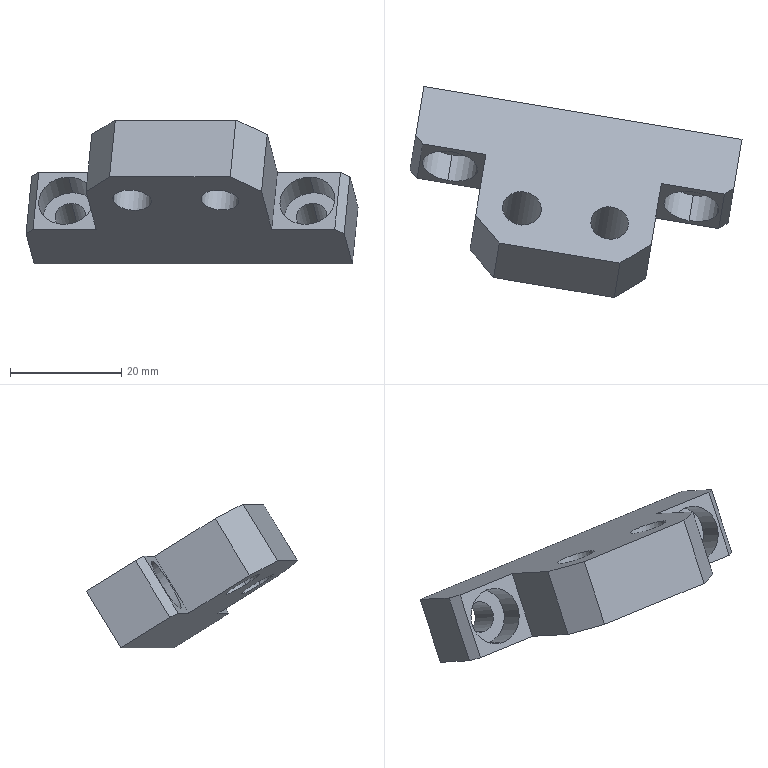Component | SolidWorks | 14AC-24-1-014-1 | 1 solid | 28 faces | box 59.71 x 37.99 x 25.9 mm | volume 12878 mm3 | plane 16 | cylinder 12 | commonest cylinder face diameters 10 x4 5.5 x4 6.8 x2 7 x2
build123d program:
from build123d import *

# Parameters (mm, degrees)
BOSS_EXTRUDE1_DEPTH                             = 12
M8X1_0_TAPPED_HOLE1_D                           = 7
CHAMFER1_SIZE                                   = 5
M5_HEX_SOCKET_HEAD_CAP_SCREW_CBORE1_D           = 5.5
M5_HEX_SOCKET_HEAD_CAP_SCREW_CBORE1_CBORE_D     = 10
M5_HEX_SOCKET_HEAD_CAP_SCREW_CBORE1_CBORE_DEPTH = 5.4
CHAMFER2_SIZE                                   = 1.5
M8_TAPPED_HOLE1_D                               = 6.8
M8_TAPPED_HOLE1_DEPTH                           = 19.75
M8_TAPPED_HOLE1_TIP                             = 2.043


with BuildPart() as part:
    # Sketch1 → Boss-Extrude1 (new body)
    with BuildSketch(Plane.XY):
        Polygon((-16, 0), (-16, 18), (16, 18), (16, 0), (29, 0), (29, -12), (-29, -12), (-29, 0), align=None)
    extrude(amount=BOSS_EXTRUDE1_DEPTH)

    # M8x1.0 Tapped Hole1 (through all)
    with Locations(Plane(origin=(-8, 10, 12), x_dir=(1, 0, 0), z_dir=(0, 0, 1))):
        with Locations((0, 0)):
            Hole(M8X1_0_TAPPED_HOLE1_D / 2)

    # Chamfer1
    chamfer1_edges = [part.edges().sort_by_distance(p)[0] for p in [
        (-16, 18, 6),
        (16, 18, 6),
    ]]
    chamfer(chamfer1_edges, length=CHAMFER1_SIZE)

    # M5 Hex Socket Head Cap Screw CBORE1 (through all)
    with Locations(Plane(origin=(-22, 0, 6), x_dir=(0, 0, 1), z_dir=(0, 1, 0))):
        with Locations((0, 0), (0, 44)):
            CounterBoreHole(M5_HEX_SOCKET_HEAD_CAP_SCREW_CBORE1_D / 2, M5_HEX_SOCKET_HEAD_CAP_SCREW_CBORE1_CBORE_D / 2, M5_HEX_SOCKET_HEAD_CAP_SCREW_CBORE1_CBORE_DEPTH)

    # Chamfer2
    chamfer2_edges = [part.edges().sort_by_distance(p)[0] for p in [
        (29, 0, 6),
        (-29, 0, 6),
    ]]
    chamfer(chamfer2_edges, length=CHAMFER2_SIZE)

    # M8 Tapped Hole1
    with Locations(Plane(origin=(8, 10, 12), x_dir=(1, 0, 0), z_dir=(0, 0, 1))):
        with Locations((0, 0)):
            Hole(M8_TAPPED_HOLE1_D / 2, depth=M8_TAPPED_HOLE1_DEPTH)
            with Locations((0, 0, -(M8_TAPPED_HOLE1_DEPTH + M8_TAPPED_HOLE1_TIP / 2))):  # 118° drill point
                Cone(0, M8_TAPPED_HOLE1_D / 2, M8_TAPPED_HOLE1_TIP, mode=Mode.SUBTRACT)


solid = part.part

# Placed as in the assembly
solid = solid.moved(Location((416.585, -110.808, -130.095), (148.871, -4.92, 8.082)))
STEP:
#1=COLOUR_RGB('',0.7922,0.8196,0.9333);
#2=FILL_AREA_STYLE_COLOUR('',#1);
#3=FILL_AREA_STYLE('',(#2));
#4=SURFACE_STYLE_FILL_AREA(#3);
#5=SURFACE_SIDE_STYLE('',(#4));
#6=SURFACE_STYLE_USAGE(.BOTH.,#5);
#7=PRESENTATION_STYLE_ASSIGNMENT((#6));
#8=CARTESIAN_POINT('',(16.524,-4.723,-4.916));
#9=VERTEX_POINT('',#8);
#10=CARTESIAN_POINT('',(16.789,-4.767,-4.916));
#11=VERTEX_POINT('',#10);
#12=CARTESIAN_POINT('',(16.657,-4.745,-4.916));
#13=DIRECTION('',(-0.08576,-0.5151,-0.8529));
#14=DIRECTION('',(0.9864,-0.1642,0.));
#15=AXIS2_PLACEMENT_3D('',#12,#13,#14);
#16=CIRCLE('',#15,0.1339);
#17=EDGE_CURVE('',#9,#11,#16,.T.);
#18=ORIENTED_EDGE('',*,*,#17,.F.);
#19=CARTESIAN_POINT('',(16.484,-4.967,-5.319));
#20=VERTEX_POINT('',#19);
#21=CARTESIAN_POINT('',(16.484,-4.967,-5.319));
#22=DIRECTION('',(-0.08576,-0.5151,-0.8529));
#23=VECTOR('',#22,39.37);
#24=LINE('',#21,#23);
#25=EDGE_CURVE('',#9,#20,#24,.T.);
#26=ORIENTED_EDGE('',*,*,#25,.T.);
#27=CARTESIAN_POINT('',(16.748,-5.011,-5.319));
#28=VERTEX_POINT('',#27);
#29=CARTESIAN_POINT('',(16.616,-4.989,-5.319));
#30=DIRECTION('',(-0.08576,-0.5151,-0.8529));
#31=DIRECTION('',(0.9864,-0.1642,0.));
#32=AXIS2_PLACEMENT_3D('',#29,#30,#31);
#33=CIRCLE('',#32,0.1339);
#34=EDGE_CURVE('',#20,#28,#33,.T.);
#35=ORIENTED_EDGE('',*,*,#34,.T.);
#36=CARTESIAN_POINT('',(16.748,-5.011,-5.319));
#37=DIRECTION('',(-0.08576,-0.5151,-0.8529));
#38=VECTOR('',#37,39.37);
#39=LINE('',#36,#38);
#40=EDGE_CURVE('',#11,#28,#39,.T.);
#41=ORIENTED_EDGE('',*,*,#40,.F.);
#42=EDGE_LOOP('',(#18,#26,#35,#41));
#43=FACE_OUTER_BOUND('',#42,.T.);
#44=CARTESIAN_POINT('',(16.616,-4.989,-5.319));
#45=DIRECTION('',(-0.08576,-0.5151,-0.8529));
#46=DIRECTION('',(0.9864,-0.1642,0.));
#47=AXIS2_PLACEMENT_3D('',#44,#45,#46);
#48=CYLINDRICAL_SURFACE('',#47,0.1339);
#49=ADVANCED_FACE('',(#43),#48,.F.);
#50=CARTESIAN_POINT('',(15.573,-4.062,-5.266));
#51=VERTEX_POINT('',#50);
#52=CARTESIAN_POINT('',(15.539,-4.264,-5.602));
#53=VERTEX_POINT('',#52);
#54=CARTESIAN_POINT('',(15.556,-4.163,-5.434));
#55=DIRECTION('',(-0.1401,-0.8413,0.5222));
#56=DIRECTION('',(-0.08576,-0.5151,-0.8529));
#57=AXIS2_PLACEMENT_3D('',#54,#55,#56);
#58=CIRCLE('',#57,0.1969);
#59=EDGE_CURVE('',#51,#53,#58,.T.);
#60=ORIENTED_EDGE('',*,*,#59,.F.);
#61=CARTESIAN_POINT('',(15.543,-4.241,-5.155));
#62=VERTEX_POINT('',#61);
#63=CARTESIAN_POINT('',(15.543,-4.241,-5.155));
#64=DIRECTION('',(-0.1401,-0.8413,0.5222));
#65=VECTOR('',#64,39.37);
#66=LINE('',#63,#65);
#67=EDGE_CURVE('',#51,#62,#66,.T.);
#68=ORIENTED_EDGE('',*,*,#67,.T.);
#69=CARTESIAN_POINT('',(15.509,-4.443,-5.491));
#70=VERTEX_POINT('',#69);
#71=CARTESIAN_POINT('',(15.526,-4.342,-5.323));
#72=DIRECTION('',(-0.1401,-0.8413,0.5222));
#73=DIRECTION('',(-0.08576,-0.5151,-0.8529));
#74=AXIS2_PLACEMENT_3D('',#71,#72,#73);
#75=CIRCLE('',#74,0.1969);
#76=EDGE_CURVE('',#62,#70,#75,.T.);
#77=ORIENTED_EDGE('',*,*,#76,.T.);
#78=CARTESIAN_POINT('',(15.509,-4.443,-5.491));
#79=DIRECTION('',(-0.1401,-0.8413,0.5222));
#80=VECTOR('',#79,39.37);
#81=LINE('',#78,#80);
#82=EDGE_CURVE('',#53,#70,#81,.T.);
#83=ORIENTED_EDGE('',*,*,#82,.F.);
#84=EDGE_LOOP('',(#60,#68,#77,#83));
#85=FACE_OUTER_BOUND('',#84,.T.);
#86=CARTESIAN_POINT('',(15.526,-4.342,-5.323));
#87=DIRECTION('',(-0.1401,-0.8413,0.5222));
#88=DIRECTION('',(-0.08576,-0.5151,-0.8529));
#89=AXIS2_PLACEMENT_3D('',#86,#87,#88);
#90=CYLINDRICAL_SURFACE('',#89,0.1969);
#91=ADVANCED_FACE('',(#85),#90,.F.);
#92=CARTESIAN_POINT('',(15.602,-3.889,-5.478));
#93=VERTEX_POINT('',#92);
#94=CARTESIAN_POINT('',(15.583,-4.,-5.662));
#95=VERTEX_POINT('',#94);
#96=CARTESIAN_POINT('',(15.593,-3.944,-5.57));
#97=DIRECTION('',(-0.1401,-0.8413,0.5222));
#98=DIRECTION('',(-0.08576,-0.5151,-0.8529));
#99=AXIS2_PLACEMENT_3D('',#96,#97,#98);
#100=CIRCLE('',#99,0.1083);
#101=EDGE_CURVE('',#93,#95,#100,.T.);
#102=ORIENTED_EDGE('',*,*,#101,.F.);
#103=CARTESIAN_POINT('',(15.565,-4.107,-5.342));
#104=VERTEX_POINT('',#103);
#105=CARTESIAN_POINT('',(15.536,-4.286,-5.231));
#106=DIRECTION('',(-0.1401,-0.8413,0.5222));
#107=VECTOR('',#106,39.37);
#108=LINE('',#105,#107);
#109=EDGE_CURVE('',#93,#104,#108,.T.);
#110=ORIENTED_EDGE('',*,*,#109,.T.);
#111=CARTESIAN_POINT('',(15.547,-4.219,-5.527));
#112=VERTEX_POINT('',#111);
#113=CARTESIAN_POINT('',(15.556,-4.163,-5.434));
#114=DIRECTION('',(-0.1401,-0.8413,0.5222));
#115=DIRECTION('',(-0.08576,-0.5151,-0.8529));
#116=AXIS2_PLACEMENT_3D('',#113,#114,#115);
#117=CIRCLE('',#116,0.1083);
#118=EDGE_CURVE('',#104,#112,#117,.T.);
#119=ORIENTED_EDGE('',*,*,#118,.T.);
#120=CARTESIAN_POINT('',(15.517,-4.398,-5.416));
#121=DIRECTION('',(-0.1401,-0.8413,0.5222));
#122=VECTOR('',#121,39.37);
#123=LINE('',#120,#122);
#124=EDGE_CURVE('',#95,#112,#123,.T.);
#125=ORIENTED_EDGE('',*,*,#124,.F.);
#126=EDGE_LOOP('',(#102,#110,#119,#125));
#127=FACE_OUTER_BOUND('',#126,.T.);
#128=CARTESIAN_POINT('',(15.526,-4.342,-5.323));
#129=DIRECTION('',(-0.1401,-0.8413,0.5222));
#130=DIRECTION('',(-0.08576,-0.5151,-0.8529));
#131=AXIS2_PLACEMENT_3D('',#128,#129,#130);
#132=CYLINDRICAL_SURFACE('',#131,0.1083);
#133=ADVANCED_FACE('',(#127),#132,.F.);
#134=CARTESIAN_POINT('',(17.282,-4.346,-5.266));
#135=VERTEX_POINT('',#134);
#136=CARTESIAN_POINT('',(17.248,-4.549,-5.602));
#137=VERTEX_POINT('',#136);
#138=CARTESIAN_POINT('',(17.265,-4.448,-5.434));
#139=DIRECTION('',(-0.1401,-0.8413,0.5222));
#140=DIRECTION('',(-0.08576,-0.5151,-0.8529));
#141=AXIS2_PLACEMENT_3D('',#138,#139,#140);
#142=CIRCLE('',#141,0.1969);
#143=EDGE_CURVE('',#135,#137,#142,.T.);
#144=ORIENTED_EDGE('',*,*,#143,.F.);
#145=CARTESIAN_POINT('',(17.252,-4.525,-5.155));
#146=VERTEX_POINT('',#145);
#147=CARTESIAN_POINT('',(17.252,-4.525,-5.155));
#148=DIRECTION('',(-0.1401,-0.8413,0.5222));
#149=VECTOR('',#148,39.37);
#150=LINE('',#147,#149);
#151=EDGE_CURVE('',#135,#146,#150,.T.);
#152=ORIENTED_EDGE('',*,*,#151,.T.);
#153=CARTESIAN_POINT('',(17.218,-4.728,-5.491));
#154=VERTEX_POINT('',#153);
#155=CARTESIAN_POINT('',(17.235,-4.626,-5.323));
#156=DIRECTION('',(-0.1401,-0.8413,0.5222));
#157=DIRECTION('',(-0.08576,-0.5151,-0.8529));
#158=AXIS2_PLACEMENT_3D('',#155,#156,#157);
#159=CIRCLE('',#158,0.1969);
#160=EDGE_CURVE('',#146,#154,#159,.T.);
#161=ORIENTED_EDGE('',*,*,#160,.T.);
#162=CARTESIAN_POINT('',(17.218,-4.728,-5.491));
#163=DIRECTION('',(-0.1401,-0.8413,0.5222));
#164=VECTOR('',#163,39.37);
#165=LINE('',#162,#164);
#166=EDGE_CURVE('',#137,#154,#165,.T.);
#167=ORIENTED_EDGE('',*,*,#166,.F.);
#168=EDGE_LOOP('',(#144,#152,#161,#167));
#169=FACE_OUTER_BOUND('',#168,.T.);
#170=CARTESIAN_POINT('',(17.235,-4.626,-5.323));
#171=DIRECTION('',(-0.1401,-0.8413,0.5222));
#172=DIRECTION('',(-0.08576,-0.5151,-0.8529));
#173=AXIS2_PLACEMENT_3D('',#170,#171,#172);
#174=CYLINDRICAL_SURFACE('',#173,0.1969);
#175=ADVANCED_FACE('',(#169),#174,.F.);
#176=CARTESIAN_POINT('',(17.311,-4.173,-5.478));
#177=VERTEX_POINT('',#176);
#178=CARTESIAN_POINT('',(17.292,-4.285,-5.662));
#179=VERTEX_POINT('',#178);
#180=CARTESIAN_POINT('',(17.301,-4.229,-5.57));
#181=DIRECTION('',(-0.1401,-0.8413,0.5222));
#182=DIRECTION('',(-0.08576,-0.5151,-0.8529));
#183=AXIS2_PLACEMENT_3D('',#180,#181,#182);
#184=CIRCLE('',#183,0.1083);
#185=EDGE_CURVE('',#177,#179,#184,.T.);
#186=ORIENTED_EDGE('',*,*,#185,.F.);
#187=CARTESIAN_POINT('',(17.274,-4.392,-5.342));
#188=VERTEX_POINT('',#187);
#189=CARTESIAN_POINT('',(17.244,-4.571,-5.231));
#190=DIRECTION('',(-0.1401,-0.8413,0.5222));
#191=VECTOR('',#190,39.37);
#192=LINE('',#189,#191);
#193=EDGE_CURVE('',#177,#188,#192,.T.);
#194=ORIENTED_EDGE('',*,*,#193,.T.);
#195=CARTESIAN_POINT('',(17.256,-4.503,-5.527));
#196=VERTEX_POINT('',#195);
#197=CARTESIAN_POINT('',(17.265,-4.448,-5.434));
#198=DIRECTION('',(-0.1401,-0.8413,0.5222));
#199=DIRECTION('',(-0.08576,-0.5151,-0.8529));
#200=AXIS2_PLACEMENT_3D('',#197,#198,#199);
#201=CIRCLE('',#200,0.1083);
#202=EDGE_CURVE('',#188,#196,#201,.T.);
#203=ORIENTED_EDGE('',*,*,#202,.T.);
#204=CARTESIAN_POINT('',(17.226,-4.682,-5.416));
#205=DIRECTION('',(-0.1401,-0.8413,0.5222));
#206=VECTOR('',#205,39.37);
#207=LINE('',#204,#206);
#208=EDGE_CURVE('',#179,#196,#207,.T.);
#209=ORIENTED_EDGE('',*,*,#208,.F.);
#210=EDGE_LOOP('',(#186,#194,#203,#209));
#211=FACE_OUTER_BOUND('',#210,.T.);
#212=CARTESIAN_POINT('',(17.235,-4.626,-5.323));
#213=DIRECTION('',(-0.1401,-0.8413,0.5222));
#214=DIRECTION('',(-0.08576,-0.5151,-0.8529));
#215=AXIS2_PLACEMENT_3D('',#212,#213,#214);
#216=CYLINDRICAL_SURFACE('',#215,0.1083);
#217=ADVANCED_FACE('',(#211),#216,.F.);
#218=CARTESIAN_POINT('',(15.899,-4.619,-4.916));
#219=VERTEX_POINT('',#218);
#220=CARTESIAN_POINT('',(16.171,-4.665,-4.916));
#221=VERTEX_POINT('',#220);
#222=CARTESIAN_POINT('',(16.035,-4.642,-4.916));
#223=DIRECTION('',(-0.08576,-0.5151,-0.8529));
#224=DIRECTION('',(0.9864,-0.1642,0.));
#225=AXIS2_PLACEMENT_3D('',#222,#223,#224);
#226=CIRCLE('',#225,0.1378);
#227=EDGE_CURVE('',#219,#221,#226,.T.);
#228=ORIENTED_EDGE('',*,*,#227,.F.);
#229=CARTESIAN_POINT('',(15.859,-4.863,-5.319));
#230=VERTEX_POINT('',#229);
#231=CARTESIAN_POINT('',(15.859,-4.863,-5.319));
#232=DIRECTION('',(-0.08576,-0.5151,-0.8529));
#233=VECTOR('',#232,39.37);
#234=LINE('',#231,#233);
#235=EDGE_CURVE('',#219,#230,#234,.T.);
#236=ORIENTED_EDGE('',*,*,#235,.T.);
#237=CARTESIAN_POINT('',(16.131,-4.908,-5.319));
#238=VERTEX_POINT('',#237);
#239=CARTESIAN_POINT('',(15.995,-4.885,-5.319));
#240=DIRECTION('',(-0.08576,-0.5151,-0.8529));
#241=DIRECTION('',(0.9864,-0.1642,0.));
#242=AXIS2_PLACEMENT_3D('',#239,#240,#241);
#243=CIRCLE('',#242,0.1378);
#244=EDGE_CURVE('',#230,#238,#243,.T.);
#245=ORIENTED_EDGE('',*,*,#244,.T.);
#246=CARTESIAN_POINT('',(16.131,-4.908,-5.319));
#247=DIRECTION('',(-0.08576,-0.5151,-0.8529));
#248=VECTOR('',#247,39.37);
#249=LINE('',#246,#248);
#250=EDGE_CURVE('',#221,#238,#249,.T.);
#251=ORIENTED_EDGE('',*,*,#250,.F.);
#252=EDGE_LOOP('',(#228,#236,#245,#251));
#253=FACE_OUTER_BOUND('',#252,.T.);
#254=CARTESIAN_POINT('',(15.995,-4.885,-5.319));
#255=DIRECTION('',(-0.08576,-0.5151,-0.8529));
#256=DIRECTION('',(0.9864,-0.1642,0.));
#257=AXIS2_PLACEMENT_3D('',#254,#255,#256);
#258=CYLINDRICAL_SURFACE('',#257,0.1378);
#259=ADVANCED_FACE('',(#253),#258,.F.);
#260=CARTESIAN_POINT('',(15.526,-4.342,-5.323));
#261=DIRECTION('',(-0.1401,-0.8413,0.5222));
#262=DIRECTION('',(-0.08576,-0.5151,-0.8529));
#263=AXIS2_PLACEMENT_3D('',#260,#261,#262);
#264=CIRCLE('',#263,0.1969);
#265=EDGE_CURVE('',#70,#62,#264,.T.);
#266=ORIENTED_EDGE('',*,*,#265,.F.);
#267=ORIENTED_EDGE('',*,*,#76,.F.);
#268=EDGE_LOOP('',(#266,#267));
#269=FACE_BOUND('',#268,.T.);
#270=CARTESIAN_POINT('',(15.78,-4.259,-5.122));
#271=VERTEX_POINT('',#270);
#272=CARTESIAN_POINT('',(15.333,-4.185,-5.122));
#273=VERTEX_POINT('',#272);
#274=CARTESIAN_POINT('',(15.275,-4.175,-5.122));
#275=DIRECTION('',(-0.9864,0.1642,0.));
#276=VECTOR('',#275,39.37);
#277=LINE('',#274,#276);
#278=EDGE_CURVE('',#271,#273,#277,.T.);
#279=ORIENTED_EDGE('',*,*,#278,.T.);
#280=CARTESIAN_POINT('',(15.292,-4.428,-5.525));
#281=VERTEX_POINT('',#280);
#282=CARTESIAN_POINT('',(15.292,-4.428,-5.525));
#283=DIRECTION('',(-0.08576,-0.5151,-0.8529));
#284=VECTOR('',#283,39.37);
#285=LINE('',#282,#284);
#286=EDGE_CURVE('',#273,#281,#285,.T.);
#287=ORIENTED_EDGE('',*,*,#286,.T.);
#288=CARTESIAN_POINT('',(15.739,-4.502,-5.525));
#289=VERTEX_POINT('',#288);
#290=CARTESIAN_POINT('',(15.234,-4.418,-5.525));
#291=DIRECTION('',(-0.9864,0.1642,0.));
#292=VECTOR('',#291,39.37);
#293=LINE('',#290,#292);
#294=EDGE_CURVE('',#289,#281,#293,.T.);
#295=ORIENTED_EDGE('',*,*,#294,.F.);
#296=CARTESIAN_POINT('',(15.739,-4.502,-5.525));
#297=DIRECTION('',(0.08576,0.5151,0.8529));
#298=VECTOR('',#297,39.37);
#299=LINE('',#296,#298);
#300=EDGE_CURVE('',#289,#271,#299,.T.);
#301=ORIENTED_EDGE('',*,*,#300,.T.);
#302=EDGE_LOOP('',(#279,#287,#295,#301));
#303=FACE_OUTER_BOUND('',#302,.T.);
#304=CARTESIAN_POINT('',(15.234,-4.418,-5.525));
#305=DIRECTION('',(0.1401,0.8413,-0.5222));
#306=DIRECTION('',(0.08576,0.5151,0.8529));
#307=AXIS2_PLACEMENT_3D('',#304,#305,#306);
#308=PLANE('',#307);
#309=ADVANCED_FACE('',(#269,#303),#308,.F.);
#310=CARTESIAN_POINT('',(15.243,-4.369,-5.556));
#311=VERTEX_POINT('',#310);
#312=CARTESIAN_POINT('',(15.3,-4.021,-5.771));
#313=VERTEX_POINT('',#312);
#314=CARTESIAN_POINT('',(15.3,-4.021,-5.771));
#315=DIRECTION('',(0.1401,0.8413,-0.5222));
#316=VECTOR('',#315,39.37);
#317=LINE('',#314,#316);
#318=EDGE_CURVE('',#311,#313,#317,.T.);
#319=ORIENTED_EDGE('',*,*,#318,.F.);
#320=CARTESIAN_POINT('',(15.283,-4.125,-5.153));
#321=VERTEX_POINT('',#320);
#322=CARTESIAN_POINT('',(15.243,-4.369,-5.556));
#323=DIRECTION('',(0.08576,0.5151,0.8529));
#324=VECTOR('',#323,39.37);
#325=LINE('',#322,#324);
#326=EDGE_CURVE('',#311,#321,#325,.T.);
#327=ORIENTED_EDGE('',*,*,#326,.T.);
#328=CARTESIAN_POINT('',(15.341,-3.778,-5.369));
#329=VERTEX_POINT('',#328);
#330=CARTESIAN_POINT('',(15.341,-3.778,-5.369));
#331=DIRECTION('',(0.1401,0.8413,-0.5222));
#332=VECTOR('',#331,39.37);
#333=LINE('',#330,#332);
#334=EDGE_CURVE('',#321,#329,#333,.T.);
#335=ORIENTED_EDGE('',*,*,#334,.T.);
#336=CARTESIAN_POINT('',(15.3,-4.021,-5.771));
#337=DIRECTION('',(0.08576,0.5151,0.8529));
#338=VECTOR('',#337,39.37);
#339=LINE('',#336,#338);
#340=EDGE_CURVE('',#313,#329,#339,.T.);
#341=ORIENTED_EDGE('',*,*,#340,.F.);
#342=EDGE_LOOP('',(#319,#327,#335,#341));
#343=FACE_OUTER_BOUND('',#342,.T.);
#344=CARTESIAN_POINT('',(15.3,-4.021,-5.771));
#345=DIRECTION('',(0.9864,-0.1642,-0.));
#346=DIRECTION('',(0.08576,0.5151,0.8529));
#347=AXIS2_PLACEMENT_3D('',#344,#345,#346);
#348=PLANE('',#347);
#349=ADVANCED_FACE('',(#343),#348,.F.);
#350=CARTESIAN_POINT('',(15.593,-3.944,-5.57));
#351=DIRECTION('',(-0.1401,-0.8413,0.5222));
#352=DIRECTION('',(-0.08576,-0.5151,-0.8529));
#353=AXIS2_PLACEMENT_3D('',#350,#351,#352);
#354=CIRCLE('',#353,0.1083);
#355=EDGE_CURVE('',#95,#93,#354,.T.);
#356=ORIENTED_EDGE('',*,*,#355,.T.);
#357=ORIENTED_EDGE('',*,*,#101,.T.);
#358=EDGE_LOOP('',(#356,#357));
#359=FACE_BOUND('',#358,.T.);
#360=CARTESIAN_POINT('',(17.301,-4.229,-5.57));
#361=DIRECTION('',(-0.1401,-0.8413,0.5222));
#362=DIRECTION('',(-0.08576,-0.5151,-0.8529));
#363=AXIS2_PLACEMENT_3D('',#360,#361,#362);
#364=CIRCLE('',#363,0.1083);
#365=EDGE_CURVE('',#179,#177,#364,.T.);
#366=ORIENTED_EDGE('',*,*,#365,.T.);
#367=ORIENTED_EDGE('',*,*,#185,.T.);
#368=EDGE_LOOP('',(#366,#367));
#369=FACE_BOUND('',#368,.T.);
#370=CARTESIAN_POINT('',(17.593,-4.153,-5.369));
#371=VERTEX_POINT('',#370);
#372=CARTESIAN_POINT('',(17.593,-4.153,-5.369));
#373=DIRECTION('',(0.9864,-0.1642,-0.));
#374=VECTOR('',#373,39.37);
#375=LINE('',#372,#374);
#376=EDGE_CURVE('',#329,#371,#375,.T.);
#377=ORIENTED_EDGE('',*,*,#376,.T.);
#378=CARTESIAN_POINT('',(17.553,-4.396,-5.771));
#379=VERTEX_POINT('',#378);
#380=CARTESIAN_POINT('',(17.553,-4.396,-5.771));
#381=DIRECTION('',(0.08576,0.5151,0.8529));
#382=VECTOR('',#381,39.37);
#383=LINE('',#380,#382);
#384=EDGE_CURVE('',#379,#371,#383,.T.);
#385=ORIENTED_EDGE('',*,*,#384,.F.);
#386=CARTESIAN_POINT('',(17.553,-4.396,-5.771));
#387=DIRECTION('',(0.9864,-0.1642,-0.));
#388=VECTOR('',#387,39.37);
#389=LINE('',#386,#388);
#390=EDGE_CURVE('',#313,#379,#389,.T.);
#391=ORIENTED_EDGE('',*,*,#390,.F.);
#392=ORIENTED_EDGE('',*,*,#340,.T.);
#393=EDGE_LOOP('',(#377,#385,#391,#392));
#394=FACE_OUTER_BOUND('',#393,.T.);
#395=CARTESIAN_POINT('',(17.553,-4.396,-5.771));
#396=DIRECTION('',(-0.1401,-0.8413,0.5222));
#397=DIRECTION('',(-0.9864,0.1642,0.));
#398=AXIS2_PLACEMENT_3D('',#395,#396,#397);
#399=PLANE('',#398);
#400=ADVANCED_FACE('',(#359,#369,#394),#399,.F.);
#401=CARTESIAN_POINT('',(17.535,-4.5,-5.153));
#402=VERTEX_POINT('',#401);
#403=CARTESIAN_POINT('',(17.527,-4.55,-5.122));
#404=DIRECTION('',(-0.1401,-0.8413,0.5222));
#405=VECTOR('',#404,39.37);
#406=LINE('',#403,#405);
#407=EDGE_CURVE('',#371,#402,#406,.T.);
#408=ORIENTED_EDGE('',*,*,#407,.T.);
#409=CARTESIAN_POINT('',(17.495,-4.744,-5.556));
#410=VERTEX_POINT('',#409);
#411=CARTESIAN_POINT('',(17.495,-4.744,-5.556));
#412=DIRECTION('',(-0.08576,-0.5151,-0.8529));
#413=VECTOR('',#412,39.37);
#414=LINE('',#411,#413);
#415=EDGE_CURVE('',#402,#410,#414,.T.);
#416=ORIENTED_EDGE('',*,*,#415,.T.);
#417=CARTESIAN_POINT('',(17.487,-4.793,-5.525));
#418=DIRECTION('',(-0.1401,-0.8413,0.5222));
#419=VECTOR('',#418,39.37);
#420=LINE('',#417,#419);
#421=EDGE_CURVE('',#379,#410,#420,.T.);
#422=ORIENTED_EDGE('',*,*,#421,.F.);
#423=ORIENTED_EDGE('',*,*,#384,.T.);
#424=EDGE_LOOP('',(#408,#416,#422,#423));
#425=FACE_OUTER_BOUND('',#424,.T.);
#426=CARTESIAN_POINT('',(17.487,-4.793,-5.525));
#427=DIRECTION('',(-0.9864,0.1642,0.));
#428=DIRECTION('',(0.1401,0.8413,-0.5222));
#429=AXIS2_PLACEMENT_3D('',#426,#427,#428);
#430=PLANE('',#429);
#431=ADVANCED_FACE('',(#425),#430,.F.);
#432=CARTESIAN_POINT('',(17.235,-4.626,-5.323));
#433=DIRECTION('',(-0.1401,-0.8413,0.5222));
#434=DIRECTION('',(-0.08576,-0.5151,-0.8529));
#435=AXIS2_PLACEMENT_3D('',#432,#433,#434);
#436=CIRCLE('',#435,0.1969);
#437=EDGE_CURVE('',#154,#146,#436,.T.);
#438=ORIENTED_EDGE('',*,*,#437,.F.);
#439=ORIENTED_EDGE('',*,*,#160,.F.);
#440=EDGE_LOOP('',(#438,#439));
#441=FACE_BOUND('',#440,.T.);
#442=CARTESIAN_POINT('',(17.428,-4.784,-5.525));
#443=VERTEX_POINT('',#442);
#444=CARTESIAN_POINT('',(16.982,-4.709,-5.525));
#445=VERTEX_POINT('',#444);
#446=CARTESIAN_POINT('',(16.982,-4.709,-5.525));
#447=DIRECTION('',(-0.9864,0.1642,0.));
#448=VECTOR('',#447,39.37);
#449=LINE('',#446,#448);
#450=EDGE_CURVE('',#443,#445,#449,.T.);
#451=ORIENTED_EDGE('',*,*,#450,.F.);
#452=CARTESIAN_POINT('',(17.469,-4.54,-5.122));
#453=VERTEX_POINT('',#452);
#454=CARTESIAN_POINT('',(17.428,-4.784,-5.525));
#455=DIRECTION('',(0.08576,0.5151,0.8529));
#456=VECTOR('',#455,39.37);
#457=LINE('',#454,#456);
#458=EDGE_CURVE('',#443,#453,#457,.T.);
#459=ORIENTED_EDGE('',*,*,#458,.T.);
#460=CARTESIAN_POINT('',(17.022,-4.466,-5.122));
#461=VERTEX_POINT('',#460);
#462=CARTESIAN_POINT('',(17.022,-4.466,-5.122));
#463=DIRECTION('',(-0.9864,0.1642,0.));
#464=VECTOR('',#463,39.37);
#465=LINE('',#462,#464);
#466=EDGE_CURVE('',#453,#461,#465,.T.);
#467=ORIENTED_EDGE('',*,*,#466,.T.);
#468=CARTESIAN_POINT('',(16.982,-4.709,-5.525));
#469=DIRECTION('',(0.08576,0.5151,0.8529));
#470=VECTOR('',#469,39.37);
#471=LINE('',#468,#470);
#472=EDGE_CURVE('',#445,#461,#471,.T.);
#473=ORIENTED_EDGE('',*,*,#472,.F.);
#474=EDGE_LOOP('',(#451,#459,#467,#473));
#475=FACE_OUTER_BOUND('',#474,.T.);
#476=CARTESIAN_POINT('',(16.982,-4.709,-5.525));
#477=DIRECTION('',(0.1401,0.8413,-0.5222));
#478=DIRECTION('',(0.9864,-0.1642,-0.));
#479=AXIS2_PLACEMENT_3D('',#476,#477,#478);
#480=PLANE('',#479);
#481=ADVANCED_FACE('',(#441,#475),#480,.F.);
#482=CARTESIAN_POINT('',(16.951,-4.897,-4.855));
#483=VERTEX_POINT('',#482);
#484=CARTESIAN_POINT('',(16.923,-5.062,-4.752));
#485=DIRECTION('',(-0.1401,-0.8413,0.5222));
#486=VECTOR('',#485,39.37);
#487=LINE('',#484,#486);
#488=EDGE_CURVE('',#461,#483,#487,.T.);
#489=ORIENTED_EDGE('',*,*,#488,.T.);
#490=CARTESIAN_POINT('',(16.91,-5.14,-5.258));
#491=VERTEX_POINT('',#490);
#492=CARTESIAN_POINT('',(16.91,-5.14,-5.258));
#493=DIRECTION('',(-0.08576,-0.5151,-0.8529));
#494=VECTOR('',#493,39.37);
#495=LINE('',#492,#494);
#496=EDGE_CURVE('',#483,#491,#495,.T.);
#497=ORIENTED_EDGE('',*,*,#496,.T.);
#498=CARTESIAN_POINT('',(16.883,-5.305,-5.155));
#499=DIRECTION('',(-0.1401,-0.8413,0.5222));
#500=VECTOR('',#499,39.37);
#501=LINE('',#498,#500);
#502=EDGE_CURVE('',#445,#491,#501,.T.);
#503=ORIENTED_EDGE('',*,*,#502,.F.);
#504=ORIENTED_EDGE('',*,*,#472,.T.);
#505=EDGE_LOOP('',(#489,#497,#503,#504));
#506=FACE_OUTER_BOUND('',#505,.T.);
#507=CARTESIAN_POINT('',(16.883,-5.305,-5.155));
#508=DIRECTION('',(-0.9864,0.1642,0.));
#509=DIRECTION('',(0.1401,0.8413,-0.5222));
#510=AXIS2_PLACEMENT_3D('',#507,#508,#509);
#511=PLANE('',#510);
#512=ADVANCED_FACE('',(#506),#511,.F.);
#513=CARTESIAN_POINT('',(16.688,-5.273,-5.155));
#514=VERTEX_POINT('',#513);
#515=CARTESIAN_POINT('',(15.834,-5.131,-5.155));
#516=VERTEX_POINT('',#515);
#517=CARTESIAN_POINT('',(15.64,-5.099,-5.155));
#518=DIRECTION('',(-0.9864,0.1642,0.));
#519=VECTOR('',#518,39.37);
#520=LINE('',#517,#519);
#521=EDGE_CURVE('',#514,#516,#520,.T.);
#522=ORIENTED_EDGE('',*,*,#521,.F.);
#523=CARTESIAN_POINT('',(16.729,-5.03,-4.752));
#524=VERTEX_POINT('',#523);
#525=CARTESIAN_POINT('',(16.688,-5.273,-5.155));
#526=DIRECTION('',(0.08576,0.5151,0.8529));
#527=VECTOR('',#526,39.37);
#528=LINE('',#525,#527);
#529=EDGE_CURVE('',#514,#524,#528,.T.);
#530=ORIENTED_EDGE('',*,*,#529,.T.);
#531=CARTESIAN_POINT('',(15.875,-4.888,-4.752));
#532=VERTEX_POINT('',#531);
#533=CARTESIAN_POINT('',(15.68,-4.855,-4.752));
#534=DIRECTION('',(-0.9864,0.1642,0.));
#535=VECTOR('',#534,39.37);
#536=LINE('',#533,#535);
#537=EDGE_CURVE('',#524,#532,#536,.T.);
#538=ORIENTED_EDGE('',*,*,#537,.T.);
#539=CARTESIAN_POINT('',(15.834,-5.131,-5.155));
#540=DIRECTION('',(-0.08576,-0.5151,-0.8529));
#541=VECTOR('',#540,39.37);
#542=LINE('',#539,#541);
#543=EDGE_CURVE('',#532,#516,#542,.T.);
#544=ORIENTED_EDGE('',*,*,#543,.T.);
#545=EDGE_LOOP('',(#522,#530,#538,#544));
#546=FACE_OUTER_BOUND('',#545,.T.);
#547=CARTESIAN_POINT('',(15.64,-5.099,-5.155));
#548=DIRECTION('',(0.1401,0.8413,-0.5222));
#549=DIRECTION('',(0.9864,-0.1642,-0.));
#550=AXIS2_PLACEMENT_3D('',#547,#548,#549);
#551=PLANE('',#550);
#552=ADVANCED_FACE('',(#546),#551,.F.);
#553=CARTESIAN_POINT('',(15.667,-4.933,-5.258));
#554=VERTEX_POINT('',#553);
#555=CARTESIAN_POINT('',(15.739,-4.502,-5.525));
#556=DIRECTION('',(0.1401,0.8413,-0.5222));
#557=VECTOR('',#556,39.37);
#558=LINE('',#555,#557);
#559=EDGE_CURVE('',#554,#289,#558,.T.);
#560=ORIENTED_EDGE('',*,*,#559,.F.);
#561=CARTESIAN_POINT('',(15.708,-4.69,-4.855));
#562=VERTEX_POINT('',#561);
#563=CARTESIAN_POINT('',(15.667,-4.933,-5.258));
#564=DIRECTION('',(0.08576,0.5151,0.8529));
#565=VECTOR('',#564,39.37);
#566=LINE('',#563,#565);
#567=EDGE_CURVE('',#554,#562,#566,.T.);
#568=ORIENTED_EDGE('',*,*,#567,.T.);
#569=CARTESIAN_POINT('',(15.78,-4.259,-5.122));
#570=DIRECTION('',(0.1401,0.8413,-0.5222));
#571=VECTOR('',#570,39.37);
#572=LINE('',#569,#571);
#573=EDGE_CURVE('',#562,#271,#572,.T.);
#574=ORIENTED_EDGE('',*,*,#573,.T.);
#575=ORIENTED_EDGE('',*,*,#300,.F.);
#576=EDGE_LOOP('',(#560,#568,#574,#575));
#577=FACE_OUTER_BOUND('',#576,.T.);
#578=CARTESIAN_POINT('',(15.739,-4.502,-5.525));
#579=DIRECTION('',(0.9864,-0.1642,-0.));
#580=DIRECTION('',(-0.1401,-0.8413,0.5222));
#581=AXIS2_PLACEMENT_3D('',#578,#579,#580);
#582=PLANE('',#581);
#583=ADVANCED_FACE('',(#577),#582,.F.);
#584=CARTESIAN_POINT('',(16.616,-4.989,-5.319));
#585=DIRECTION('',(-0.08576,-0.5151,-0.8529));
#586=DIRECTION('',(0.9864,-0.1642,0.));
#587=AXIS2_PLACEMENT_3D('',#584,#585,#586);
#588=CIRCLE('',#587,0.1339);
#589=EDGE_CURVE('',#28,#20,#588,.T.);
#590=ORIENTED_EDGE('',*,*,#589,.F.);
#591=ORIENTED_EDGE('',*,*,#34,.F.);
#592=EDGE_LOOP('',(#590,#591));
#593=FACE_BOUND('',#592,.T.);
#594=CARTESIAN_POINT('',(15.995,-4.885,-5.319));
#595=DIRECTION('',(-0.08576,-0.5151,-0.8529));
#596=DIRECTION('',(0.9864,-0.1642,0.));
#597=AXIS2_PLACEMENT_3D('',#594,#595,#596);
#598=CIRCLE('',#597,0.1378);
#599=EDGE_CURVE('',#238,#230,#598,.T.);
#600=ORIENTED_EDGE('',*,*,#599,.F.);
#601=ORIENTED_EDGE('',*,*,#244,.F.);
#602=EDGE_LOOP('',(#600,#601));
#603=FACE_BOUND('',#602,.T.);
#604=ORIENTED_EDGE('',*,*,#421,.T.);
#605=CARTESIAN_POINT('',(16.819,-5.15,-5.242));
#606=DIRECTION('',(-0.7966,-0.4787,0.3692));
#607=VECTOR('',#606,39.37);
#608=LINE('',#605,#607);
#609=EDGE_CURVE('',#410,#443,#608,.T.);
#610=ORIENTED_EDGE('',*,*,#609,.T.);
#611=ORIENTED_EDGE('',*,*,#450,.T.);
#612=ORIENTED_EDGE('',*,*,#502,.T.);
#613=CARTESIAN_POINT('',(16.844,-5.18,-5.227));
#614=DIRECTION('',(-0.7966,-0.4787,0.3692));
#615=VECTOR('',#614,39.37);
#616=LINE('',#613,#615);
#617=EDGE_CURVE('',#491,#514,#616,.T.);
#618=ORIENTED_EDGE('',*,*,#617,.T.);
#619=ORIENTED_EDGE('',*,*,#521,.T.);
#620=CARTESIAN_POINT('',(15.717,-4.992,-5.227));
#621=DIRECTION('',(-0.5985,0.711,-0.3692));
#622=VECTOR('',#621,39.37);
#623=LINE('',#620,#622);
#624=EDGE_CURVE('',#516,#554,#623,.T.);
#625=ORIENTED_EDGE('',*,*,#624,.T.);
#626=ORIENTED_EDGE('',*,*,#559,.T.);
#627=ORIENTED_EDGE('',*,*,#294,.T.);
#628=CARTESIAN_POINT('',(15.751,-4.972,-5.242));
#629=DIRECTION('',(-0.5985,0.711,-0.3692));
#630=VECTOR('',#629,39.37);
#631=LINE('',#628,#630);
#632=EDGE_CURVE('',#281,#311,#631,.T.);
#633=ORIENTED_EDGE('',*,*,#632,.T.);
#634=ORIENTED_EDGE('',*,*,#318,.T.);
#635=ORIENTED_EDGE('',*,*,#390,.T.);
#636=EDGE_LOOP('',(#604,#610,#611,#612,#618,#619,#625,#626,#627,#633,#634,#635));
#637=FACE_OUTER_BOUND('',#636,.T.);
#638=CARTESIAN_POINT('',(16.36,-4.606,-5.525));
#639=DIRECTION('',(-0.08576,-0.5151,-0.8529));
#640=DIRECTION('',(0.9864,-0.1642,-0.));
#641=AXIS2_PLACEMENT_3D('',#638,#639,#640);
#642=PLANE('',#641);
#643=ADVANCED_FACE('',(#593,#603,#637),#642,.T.);
#644=CARTESIAN_POINT('',(16.657,-4.745,-4.916));
#645=DIRECTION('',(-0.08576,-0.5151,-0.8529));
#646=DIRECTION('',(0.9864,-0.1642,0.));
#647=AXIS2_PLACEMENT_3D('',#644,#645,#646);
#648=CIRCLE('',#647,0.1339);
#649=EDGE_CURVE('',#11,#9,#648,.T.);
#650=ORIENTED_EDGE('',*,*,#649,.T.);
#651=ORIENTED_EDGE('',*,*,#17,.T.);
#652=EDGE_LOOP('',(#650,#651));
#653=FACE_BOUND('',#652,.T.);
#654=CARTESIAN_POINT('',(16.035,-4.642,-4.916));
#655=DIRECTION('',(-0.08576,-0.5151,-0.8529));
#656=DIRECTION('',(0.9864,-0.1642,0.));
#657=AXIS2_PLACEMENT_3D('',#654,#655,#656);
#658=CIRCLE('',#657,0.1378);
#659=EDGE_CURVE('',#221,#219,#658,.T.);
#660=ORIENTED_EDGE('',*,*,#659,.T.);
#661=ORIENTED_EDGE('',*,*,#227,.T.);
#662=EDGE_LOOP('',(#660,#661));
#663=FACE_BOUND('',#662,.T.);
#664=ORIENTED_EDGE('',*,*,#466,.F.);
#665=CARTESIAN_POINT('',(17.469,-4.54,-5.122));
#666=DIRECTION('',(0.7966,0.4787,-0.3692));
#667=VECTOR('',#666,39.37);
#668=LINE('',#665,#667);
#669=EDGE_CURVE('',#453,#402,#668,.T.);
#670=ORIENTED_EDGE('',*,*,#669,.T.);
#671=ORIENTED_EDGE('',*,*,#407,.F.);
#672=ORIENTED_EDGE('',*,*,#376,.F.);
#673=ORIENTED_EDGE('',*,*,#334,.F.);
#674=CARTESIAN_POINT('',(15.283,-4.125,-5.153));
#675=DIRECTION('',(0.5985,-0.711,0.3692));
#676=VECTOR('',#675,39.37);
#677=LINE('',#674,#676);
#678=EDGE_CURVE('',#321,#273,#677,.T.);
#679=ORIENTED_EDGE('',*,*,#678,.T.);
#680=ORIENTED_EDGE('',*,*,#278,.F.);
#681=ORIENTED_EDGE('',*,*,#573,.F.);
#682=CARTESIAN_POINT('',(15.708,-4.69,-4.855));
#683=DIRECTION('',(0.5985,-0.711,0.3692));
#684=VECTOR('',#683,39.37);
#685=LINE('',#682,#684);
#686=EDGE_CURVE('',#562,#532,#685,.T.);
#687=ORIENTED_EDGE('',*,*,#686,.T.);
#688=ORIENTED_EDGE('',*,*,#537,.F.);
#689=CARTESIAN_POINT('',(16.729,-5.03,-4.752));
#690=DIRECTION('',(0.7966,0.4787,-0.3692));
#691=VECTOR('',#690,39.37);
#692=LINE('',#689,#691);
#693=EDGE_CURVE('',#524,#483,#692,.T.);
#694=ORIENTED_EDGE('',*,*,#693,.T.);
#695=ORIENTED_EDGE('',*,*,#488,.F.);
#696=EDGE_LOOP('',(#664,#670,#671,#672,#673,#679,#680,#681,#687,#688,#694,#695));
#697=FACE_OUTER_BOUND('',#696,.T.);
#698=CARTESIAN_POINT('',(16.401,-4.363,-5.122));
#699=DIRECTION('',(-0.08576,-0.5151,-0.8529));
#700=DIRECTION('',(0.9864,-0.1642,-0.));
#701=AXIS2_PLACEMENT_3D('',#698,#699,#700);
#702=PLANE('',#701);
#703=ADVANCED_FACE('',(#653,#663,#697),#702,.F.);
#704=ORIENTED_EDGE('',*,*,#235,.F.);
#705=ORIENTED_EDGE('',*,*,#659,.F.);
#706=ORIENTED_EDGE('',*,*,#250,.T.);
#707=ORIENTED_EDGE('',*,*,#599,.T.);
#708=EDGE_LOOP('',(#704,#705,#706,#707));
#709=FACE_OUTER_BOUND('',#708,.T.);
#710=CARTESIAN_POINT('',(15.995,-4.885,-5.319));
#711=DIRECTION('',(-0.08576,-0.5151,-0.8529));
#712=DIRECTION('',(0.9864,-0.1642,0.));
#713=AXIS2_PLACEMENT_3D('',#710,#711,#712);
#714=CYLINDRICAL_SURFACE('',#713,0.1378);
#715=ADVANCED_FACE('',(#709),#714,.F.);
#716=ORIENTED_EDGE('',*,*,#617,.F.);
#717=ORIENTED_EDGE('',*,*,#496,.F.);
#718=ORIENTED_EDGE('',*,*,#693,.F.);
#719=ORIENTED_EDGE('',*,*,#529,.F.);
#720=EDGE_LOOP('',(#716,#717,#718,#719));
#721=FACE_OUTER_BOUND('',#720,.T.);
#722=CARTESIAN_POINT('',(16.688,-5.273,-5.155));
#723=DIRECTION('',(-0.5985,0.711,-0.3692));
#724=DIRECTION('',(0.08576,0.5151,0.8529));
#725=AXIS2_PLACEMENT_3D('',#722,#723,#724);
#726=PLANE('',#725);
#727=ADVANCED_FACE('',(#721),#726,.F.);
#728=ORIENTED_EDGE('',*,*,#624,.F.);
#729=ORIENTED_EDGE('',*,*,#543,.F.);
#730=ORIENTED_EDGE('',*,*,#686,.F.);
#731=ORIENTED_EDGE('',*,*,#567,.F.);
#732=EDGE_LOOP('',(#728,#729,#730,#731));
#733=FACE_OUTER_BOUND('',#732,.T.);
#734=CARTESIAN_POINT('',(15.667,-4.933,-5.258));
#735=DIRECTION('',(0.7966,0.4787,-0.3692));
#736=DIRECTION('',(0.08576,0.5151,0.8529));
#737=AXIS2_PLACEMENT_3D('',#734,#735,#736);
#738=PLANE('',#737);
#739=ADVANCED_FACE('',(#733),#738,.F.);
#740=ORIENTED_EDGE('',*,*,#193,.F.);
#741=ORIENTED_EDGE('',*,*,#365,.F.);
#742=ORIENTED_EDGE('',*,*,#208,.T.);
#743=CARTESIAN_POINT('',(17.265,-4.448,-5.434));
#744=DIRECTION('',(-0.1401,-0.8413,0.5222));
#745=DIRECTION('',(-0.08576,-0.5151,-0.8529));
#746=AXIS2_PLACEMENT_3D('',#743,#744,#745);
#747=CIRCLE('',#746,0.1083);
#748=EDGE_CURVE('',#196,#188,#747,.T.);
#749=ORIENTED_EDGE('',*,*,#748,.T.);
#750=EDGE_LOOP('',(#740,#741,#742,#749));
#751=FACE_OUTER_BOUND('',#750,.T.);
#752=CARTESIAN_POINT('',(17.235,-4.626,-5.323));
#753=DIRECTION('',(-0.1401,-0.8413,0.5222));
#754=DIRECTION('',(-0.08576,-0.5151,-0.8529));
#755=AXIS2_PLACEMENT_3D('',#752,#753,#754);
#756=CYLINDRICAL_SURFACE('',#755,0.1083);
#757=ADVANCED_FACE('',(#751),#756,.F.);
#758=ORIENTED_EDGE('',*,*,#748,.F.);
#759=ORIENTED_EDGE('',*,*,#202,.F.);
#760=EDGE_LOOP('',(#758,#759));
#761=FACE_BOUND('',#760,.T.);
#762=CARTESIAN_POINT('',(17.265,-4.448,-5.434));
#763=DIRECTION('',(-0.1401,-0.8413,0.5222));
#764=DIRECTION('',(-0.08576,-0.5151,-0.8529));
#765=AXIS2_PLACEMENT_3D('',#762,#763,#764);
#766=CIRCLE('',#765,0.1969);
#767=EDGE_CURVE('',#137,#135,#766,.T.);
#768=ORIENTED_EDGE('',*,*,#767,.T.);
#769=ORIENTED_EDGE('',*,*,#143,.T.);
#770=EDGE_LOOP('',(#768,#769));
#771=FACE_OUTER_BOUND('',#770,.T.);
#772=CARTESIAN_POINT('',(17.372,-4.465,-5.434));
#773=DIRECTION('',(0.1401,0.8413,-0.5222));
#774=DIRECTION('',(0.08576,0.5151,0.8529));
#775=AXIS2_PLACEMENT_3D('',#772,#773,#774);
#776=PLANE('',#775);
#777=ADVANCED_FACE('',(#761,#771),#776,.F.);
#778=ORIENTED_EDGE('',*,*,#151,.F.);
#779=ORIENTED_EDGE('',*,*,#767,.F.);
#780=ORIENTED_EDGE('',*,*,#166,.T.);
#781=ORIENTED_EDGE('',*,*,#437,.T.);
#782=EDGE_LOOP('',(#778,#779,#780,#781));
#783=FACE_OUTER_BOUND('',#782,.T.);
#784=CARTESIAN_POINT('',(17.235,-4.626,-5.323));
#785=DIRECTION('',(-0.1401,-0.8413,0.5222));
#786=DIRECTION('',(-0.08576,-0.5151,-0.8529));
#787=AXIS2_PLACEMENT_3D('',#784,#785,#786);
#788=CYLINDRICAL_SURFACE('',#787,0.1969);
#789=ADVANCED_FACE('',(#783),#788,.F.);
#790=ORIENTED_EDGE('',*,*,#109,.F.);
#791=ORIENTED_EDGE('',*,*,#355,.F.);
#792=ORIENTED_EDGE('',*,*,#124,.T.);
#793=CARTESIAN_POINT('',(15.556,-4.163,-5.434));
#794=DIRECTION('',(-0.1401,-0.8413,0.5222));
#795=DIRECTION('',(-0.08576,-0.5151,-0.8529));
#796=AXIS2_PLACEMENT_3D('',#793,#794,#795);
#797=CIRCLE('',#796,0.1083);
#798=EDGE_CURVE('',#112,#104,#797,.T.);
#799=ORIENTED_EDGE('',*,*,#798,.T.);
#800=EDGE_LOOP('',(#790,#791,#792,#799));
#801=FACE_OUTER_BOUND('',#800,.T.);
#802=CARTESIAN_POINT('',(15.526,-4.342,-5.323));
#803=DIRECTION('',(-0.1401,-0.8413,0.5222));
#804=DIRECTION('',(-0.08576,-0.5151,-0.8529));
#805=AXIS2_PLACEMENT_3D('',#802,#803,#804);
#806=CYLINDRICAL_SURFACE('',#805,0.1083);
#807=ADVANCED_FACE('',(#801),#806,.F.);
#808=ORIENTED_EDGE('',*,*,#798,.F.);
#809=ORIENTED_EDGE('',*,*,#118,.F.);
#810=EDGE_LOOP('',(#808,#809));
#811=FACE_BOUND('',#810,.T.);
#812=CARTESIAN_POINT('',(15.556,-4.163,-5.434));
#813=DIRECTION('',(-0.1401,-0.8413,0.5222));
#814=DIRECTION('',(-0.08576,-0.5151,-0.8529));
#815=AXIS2_PLACEMENT_3D('',#812,#813,#814);
#816=CIRCLE('',#815,0.1969);
#817=EDGE_CURVE('',#53,#51,#816,.T.);
#818=ORIENTED_EDGE('',*,*,#817,.T.);
#819=ORIENTED_EDGE('',*,*,#59,.T.);
#820=EDGE_LOOP('',(#818,#819));
#821=FACE_OUTER_BOUND('',#820,.T.);
#822=CARTESIAN_POINT('',(15.663,-4.181,-5.434));
#823=DIRECTION('',(0.1401,0.8413,-0.5222));
#824=DIRECTION('',(0.08576,0.5151,0.8529));
#825=AXIS2_PLACEMENT_3D('',#822,#823,#824);
#826=PLANE('',#825);
#827=ADVANCED_FACE('',(#811,#821),#826,.F.);
#828=ORIENTED_EDGE('',*,*,#67,.F.);
#829=ORIENTED_EDGE('',*,*,#817,.F.);
#830=ORIENTED_EDGE('',*,*,#82,.T.);
#831=ORIENTED_EDGE('',*,*,#265,.T.);
#832=EDGE_LOOP('',(#828,#829,#830,#831));
#833=FACE_OUTER_BOUND('',#832,.T.);
#834=CARTESIAN_POINT('',(15.526,-4.342,-5.323));
#835=DIRECTION('',(-0.1401,-0.8413,0.5222));
#836=DIRECTION('',(-0.08576,-0.5151,-0.8529));
#837=AXIS2_PLACEMENT_3D('',#834,#835,#836);
#838=CYLINDRICAL_SURFACE('',#837,0.1969);
#839=ADVANCED_FACE('',(#833),#838,.F.);
#840=ORIENTED_EDGE('',*,*,#609,.F.);
#841=ORIENTED_EDGE('',*,*,#415,.F.);
#842=ORIENTED_EDGE('',*,*,#669,.F.);
#843=ORIENTED_EDGE('',*,*,#458,.F.);
#844=EDGE_LOOP('',(#840,#841,#842,#843));
#845=FACE_OUTER_BOUND('',#844,.T.);
#846=CARTESIAN_POINT('',(17.428,-4.784,-5.525));
#847=DIRECTION('',(-0.5985,0.711,-0.3692));
#848=DIRECTION('',(0.08576,0.5151,0.8529));
#849=AXIS2_PLACEMENT_3D('',#846,#847,#848);
#850=PLANE('',#849);
#851=ADVANCED_FACE('',(#845),#850,.F.);
#852=ORIENTED_EDGE('',*,*,#632,.F.);
#853=ORIENTED_EDGE('',*,*,#286,.F.);
#854=ORIENTED_EDGE('',*,*,#678,.F.);
#855=ORIENTED_EDGE('',*,*,#326,.F.);
#856=EDGE_LOOP('',(#852,#853,#854,#855));
#857=FACE_OUTER_BOUND('',#856,.T.);
#858=CARTESIAN_POINT('',(15.243,-4.369,-5.556));
#859=DIRECTION('',(0.7966,0.4787,-0.3692));
#860=DIRECTION('',(0.08576,0.5151,0.8529));
#861=AXIS2_PLACEMENT_3D('',#858,#859,#860);
#862=PLANE('',#861);
#863=ADVANCED_FACE('',(#857),#862,.F.);
#864=ORIENTED_EDGE('',*,*,#25,.F.);
#865=ORIENTED_EDGE('',*,*,#649,.F.);
#866=ORIENTED_EDGE('',*,*,#40,.T.);
#867=ORIENTED_EDGE('',*,*,#589,.T.);
#868=EDGE_LOOP('',(#864,#865,#866,#867));
#869=FACE_OUTER_BOUND('',#868,.T.);
#870=CARTESIAN_POINT('',(16.616,-4.989,-5.319));
#871=DIRECTION('',(-0.08576,-0.5151,-0.8529));
#872=DIRECTION('',(0.9864,-0.1642,0.));
#873=AXIS2_PLACEMENT_3D('',#870,#871,#872);
#874=CYLINDRICAL_SURFACE('',#873,0.1339);
#875=ADVANCED_FACE('',(#869),#874,.F.);
#876=CLOSED_SHELL('',(#49,#91,#133,#175,#217,#259,#309,#349,#400,#431,#481,#512,#552,#583,#643,#703,#715,#727,#739,#757,#777,#789,#807,#827,#839,#851,#863,#875));
#877=MANIFOLD_SOLID_BREP('',#876);
#878=STYLED_ITEM('',(#7),#877);
#879=(LENGTH_UNIT()NAMED_UNIT(*)SI_UNIT($,.METRE.));
#880=LENGTH_MEASURE_WITH_UNIT(LENGTH_MEASURE(0.0254),#879);
#881=DIMENSIONAL_EXPONENTS(1.,0.,0.,0.,0.,0.,0.);
#882=(CONVERSION_BASED_UNIT('',#880)LENGTH_UNIT()NAMED_UNIT(#881));
#883=UNCERTAINTY_MEASURE_WITH_UNIT(LENGTH_MEASURE(0.00001),#882,'','');
#884=(NAMED_UNIT(*)PLANE_ANGLE_UNIT()SI_UNIT($,.RADIAN.));
#885=(NAMED_UNIT(*)SI_UNIT($,.STERADIAN.)SOLID_ANGLE_UNIT());
#886=(GEOMETRIC_REPRESENTATION_CONTEXT(3)GLOBAL_UNCERTAINTY_ASSIGNED_CONTEXT((#883))GLOBAL_UNIT_ASSIGNED_CONTEXT((#882,#884,#885))REPRESENTATION_CONTEXT('',''));
#887=MECHANICAL_DESIGN_GEOMETRIC_PRESENTATION_REPRESENTATION('',(#878),#886);
#888=PRESENTATION_LAYER_ASSIGNMENT('','',(#878));
#889=CARTESIAN_POINT('',(0.,0.,0.));
#890=DIRECTION('',(0.,0.,1.));
#891=DIRECTION('',(1.,0.,0.));
#892=AXIS2_PLACEMENT_3D('',#889,#890,#891);
#893=(LENGTH_UNIT()NAMED_UNIT(*)SI_UNIT($,.METRE.));
#894=LENGTH_MEASURE_WITH_UNIT(LENGTH_MEASURE(0.0254),#893);
#895=DIMENSIONAL_EXPONENTS(1.,0.,0.,0.,0.,0.,0.);
#896=(CONVERSION_BASED_UNIT('',#894)LENGTH_UNIT()NAMED_UNIT(#895));
#897=UNCERTAINTY_MEASURE_WITH_UNIT(LENGTH_MEASURE(0.00001),#896,'','');
#898=(NAMED_UNIT(*)PLANE_ANGLE_UNIT()SI_UNIT($,.RADIAN.));
#899=(NAMED_UNIT(*)SI_UNIT($,.STERADIAN.)SOLID_ANGLE_UNIT());
#900=(GEOMETRIC_REPRESENTATION_CONTEXT(3)GLOBAL_UNCERTAINTY_ASSIGNED_CONTEXT((#897))GLOBAL_UNIT_ASSIGNED_CONTEXT((#896,#898,#899))REPRESENTATION_CONTEXT('',''));
#901=ADVANCED_BREP_SHAPE_REPRESENTATION('',(#877,#892),#900);